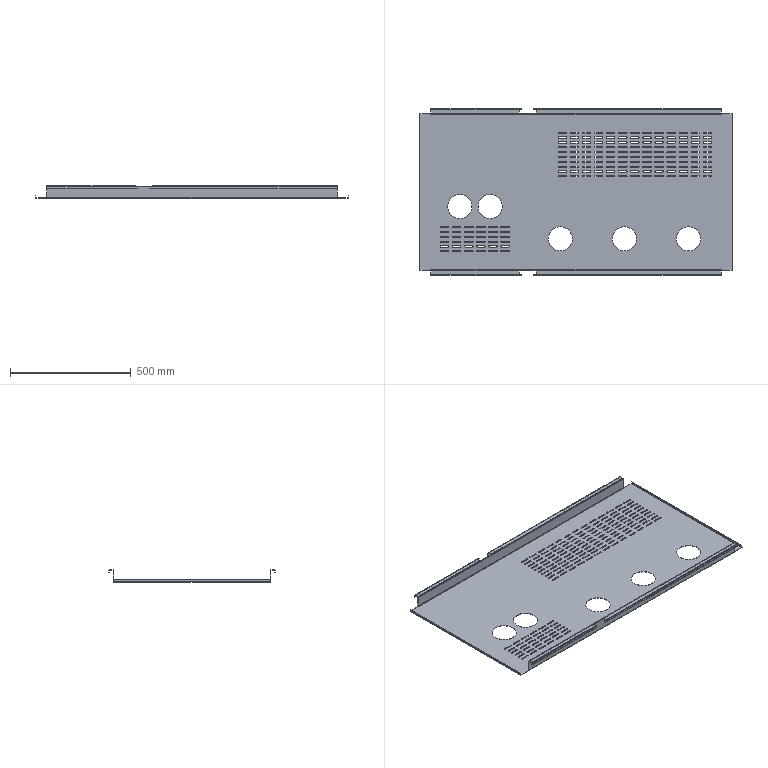Component | SolidWorks | BottomPlate4-1 | 1 solid | 966 faces | volume 1434049 mm3 | cylinder 528 | plane 438 | commonest cylinder face diameters 5 x498 100 x10 6 x10 3 x10